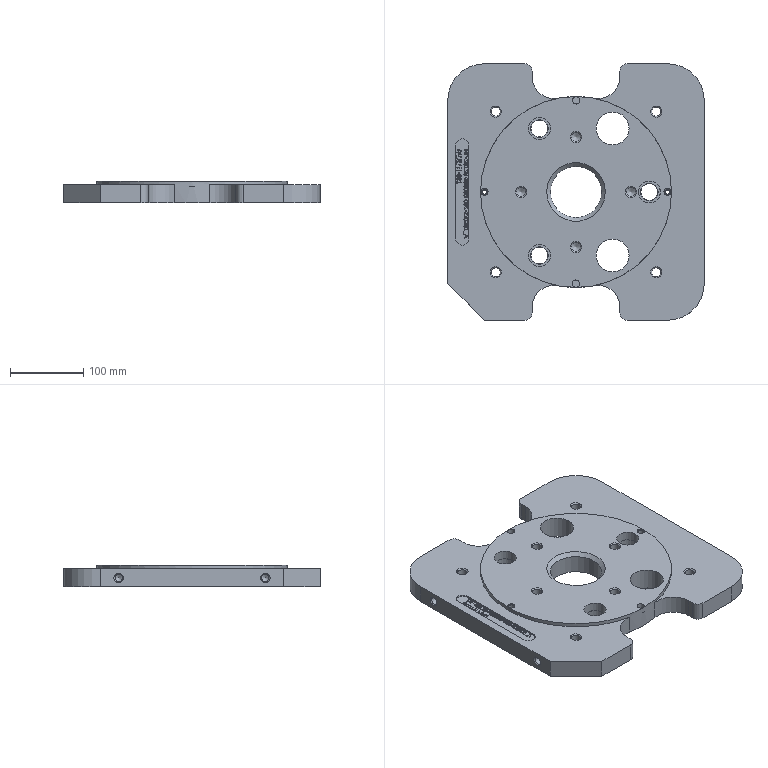CAM job | NX | mm | 3-axis | 4 set-ups | 62 operations | part box 350 x 350 x 30
set-up 1
1. Planar Milling | Mill Mill5 LX-D12 | PLANAR_MILLING_1 | path 52963.207 mm | 12.995 min
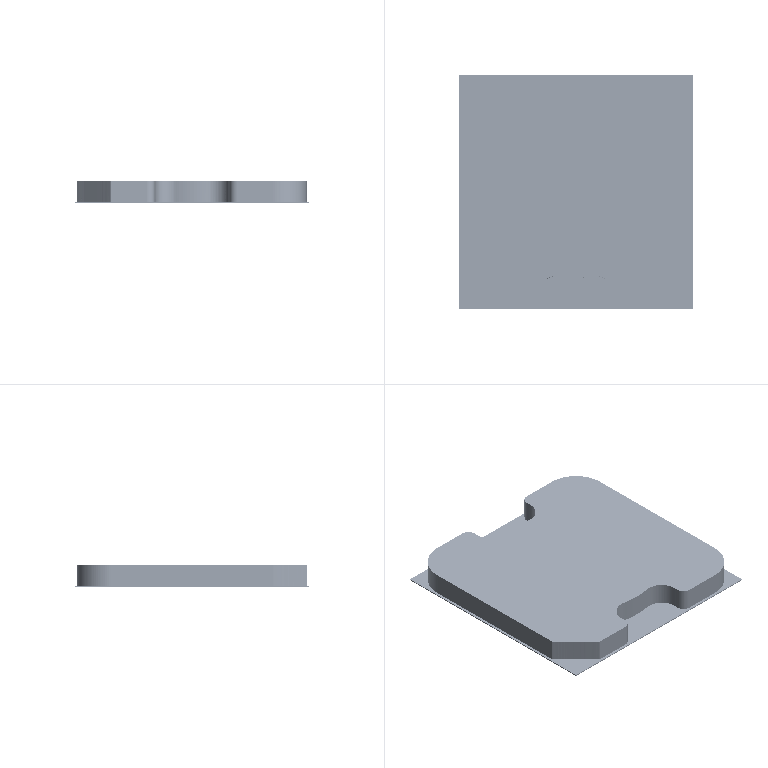2. Drilling | Mill MillChamfer DXZ-D6A90 | DRILLING_2 | path 472.41 mm | 0.166 min
3. Drilling | Drill DrillStandard ZT-D9.9 | DRILLING_3 | path 1885.71 mm | 2.188 min
4. Cavity Milling | Mill Mill5 LX-D12 | CAVITY_MILLING_4 | path 120910.672 mm | 30.327 min
5. Cavity Milling | Mill Mill5 LX-D12 | CAVITY_MILLING_5 | path 21409.338 mm | 17.162 min
set-up 2
6. Face Milling | Mill Mill5 E50R0.8 | FACE_MILLING_6 | path 20984.363 mm | 9.761 min
7. Planar Milling | Mill Mill5 LX-D12 | PLANAR_MILLING_7 | path 17688.841 mm | 4.155 min
8. Planar Milling | Mill Mill5 LX-D12 | PLANAR_MILLING_8 | path 2612.83 mm | 0.6251 min
9. Planar Milling | Mill Mill5 LX-D12 | PLANAR_MILLING_9 | path 3553.203 mm | 0.8071 min
10. Drilling | Mill MillChamfer DXZ-D6A90 | DRILLING_10 | path 344 mm | 0.1669 min
11. Drilling | Mill MillChamfer DXZ-D6A90 | DRILLING_11 | path 845.609 mm | 0.3496 min
12. Drilling | Drill DrillStandard ZT-D5.5 | DRILLING_12 | path 1324 mm | 1.534 min
13. Drilling | Drill DrillStandard ZT-D10.5 | DRILLING_13 | path 2815.498 mm | 3.098 min
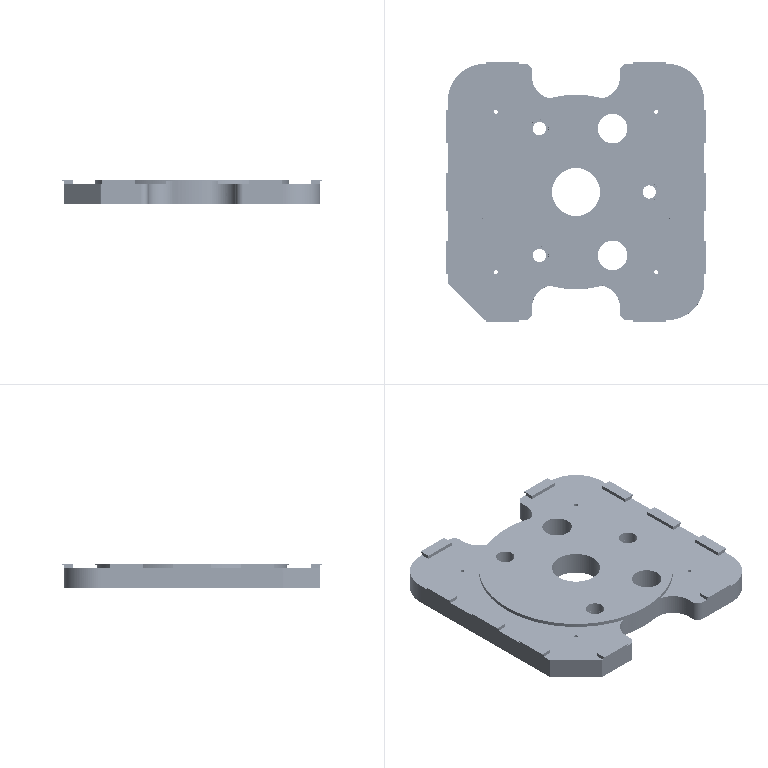14. Cylinder Milling | Mill Mill5 LX-D10 | CYLINDER_MILLING_14 | path 2394.779 mm | 1.918 min
15. Face Milling | Mill Mill5 E50R0.8 | FACE_MILLING_15 | path 6441 mm | 8.011 min
16. Cylinder Milling | Mill Mill5 LX-D10J | CYLINDER_MILLING_16 | path 1842.35 mm | 2.364 min
17. Planar Milling | Mill Mill5 LX-D12J | PLANAR_MILLING_17 | path 901.756 mm | 0.5999 min
18. Planar Milling | Mill Mill5 LX-D12J | PLANAR_MILLING_18 | path 3088.498 mm | 3.698 min
19. Thread Milling | Drill DrillThreadMill ST12X1.75-D10 | THREAD_MILLING_19 | path 4743.054 mm | 6.86 min
20. Thread Milling | Drill DrillThreadMill ST12X1.75-D10 | THREAD_MILLING_20 | path 1740.533 mm | 1.698 min
21. Volume Based 2.5D Milling | Mill MillChamfer DJ-D10A90 | VOLUME_BASED_2.5D_MILLING_21 | path 1306.051 mm | 0.5446 min
22. Fixed-axis Surface Contouring | Mill MillChamfer DJ-D10A90 | FIXED-AXIS_SURFACE_CONTOURING_22 | path 3704.367 mm | 2.34 min
23. Planar Milling | Mill Mill5 LX-D12J | PLANAR_MILLING_23 | path 13798.065 mm | 5.494 min
set-up 3
24. Face Milling | Mill Mill5 E50R0.8 | FACE_MILLING_24 | path 10729.483 mm | 5.016 min
25. Cavity Milling | Mill Mill5 LX-D12 | CAVITY_MILLING_25 | path 63705.335 mm | 15.092 min
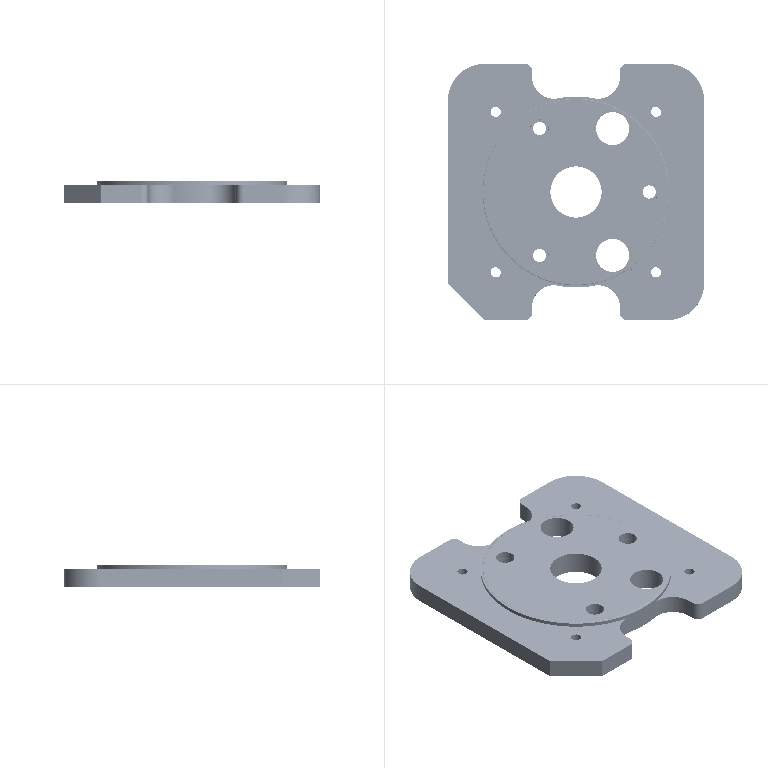26. Cylinder Milling | Mill Mill5 LX-D12 | CYLINDER_MILLING_26 | path 3593.116 mm | 3.95 min
27. Cylinder Milling | Mill Mill5 LX-D12 | CYLINDER_MILLING_27 | path 3455.636 mm | 3.694 min
28. Cylinder Milling | Mill Mill5 LX-D12 | CYLINDER_MILLING_28 | path 1601.601 mm | 1.295 min
29. Drilling | Mill MillChamfer DXZ-D6A90 | DRILLING_29 | path 739.906 mm | 0.3116 min
30. Drilling | Drill DrillStandard ZT-D11.5 | DRILLING_30 | path 1805.513 mm | 2.375 min
31. Drilling | Drill DrillStandard ZT-D7.5 | DRILLING_31 | path 598 mm | 0.7536 min
32. Cylinder Milling | Mill Mill5 LX-D8 | CYLINDER_MILLING_32 | path 2246.266 mm | 2.14 min
33. Volume Based 2.5D Milling | Mill Mill5 LX-D8 | VOLUME_BASED_2.5D_MILLING_33 | path 2636.289 mm | 0.7371 min
34. Cylinder Milling | Mill Mill5 LX-D6 | CYLINDER_MILLING_34 | path 689.766 mm | 0.4379 min
35. Cylinder Milling | Mill Mill5 LX-D6 | CYLINDER_MILLING_35 | path 721.625 mm | 0.5024 min
36. Face Milling | Mill Mill5 E50R0.8 | FACE_MILLING_36 | path 3024.894 mm | 3.736 min
37. Cylinder Milling | Mill Mill5 LX-D6J | CYLINDER_MILLING_37 | path 622.291 mm | 0.6705 min
38. Cylinder Milling | Mill Mill5 LX-D6J | CYLINDER_MILLING_38 | path 620.498 mm | 0.7172 min
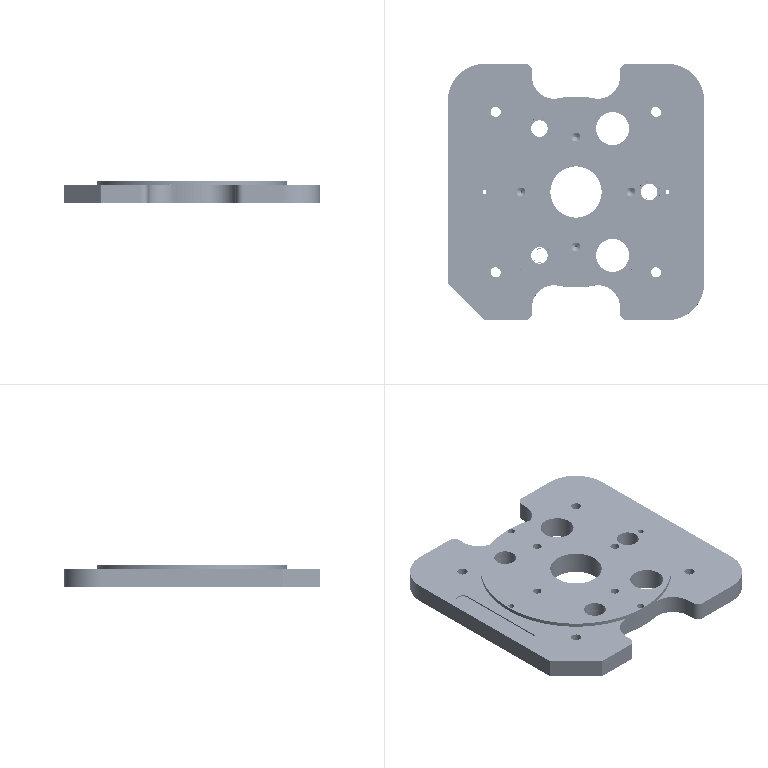39. Cylinder Milling | Mill Mill5 LX-D8J | CYLINDER_MILLING_39 | path 2076.707 mm | 3.799 min
40. Volume Based 2.5D Milling | Mill Mill5 LX-D8J | VOLUME_BASED_2.5D_MILLING_40 | path 817.628 mm | 1.033 min
41. Volume Based 2.5D Milling | Mill Mill5 LX-D8J | VOLUME_BASED_2.5D_MILLING_41 | path 348.948 mm | 0.3741 min
42. Volume Based 2.5D Milling | Mill Mill5 LX-D12J | VOLUME_BASED_2.5D_MILLING_42 | path 11476.04 mm | 12.766 min
43. Volume Based 2.5D Milling | Mill Mill5 LX-D12J | VOLUME_BASED_2.5D_MILLING_43 | path 918.725 mm | 0.9751 min
44. Cylinder Milling | Mill Mill5 LX-D12J | CYLINDER_MILLING_44 | path 1948.545 mm | 3.739 min
45. Cylinder Milling | Mill Mill5 LX-D12J | CYLINDER_MILLING_45 | path 1934.602 mm | 3.527 min
46. Cylinder Milling | Mill Mill5 LX-D12J | CYLINDER_MILLING_46 | path 1094.948 mm | 1.218 min
47. Planar Milling | Mill Mill5 LX-D12J | PLANAR_MILLING_47 | path 515.038 mm | 0.487 min
48. Volume Based 2.5D Milling | Mill MillChamfer DJ-D12A90 | VOLUME_BASED_2.5D_MILLING_48 | path 961.193 mm | 0.9166 min
49. Volume Based 2.5D Milling | Mill MillChamfer DJ-D12A90 | VOLUME_BASED_2.5D_MILLING_49 | path 1365.965 mm | 0.9176 min
50. Volume Based 2.5D Milling | Mill MillChamfer DJ-D12A90 | VOLUME_BASED_2.5D_MILLING_50 | path 737.716 mm | 0.4306 min
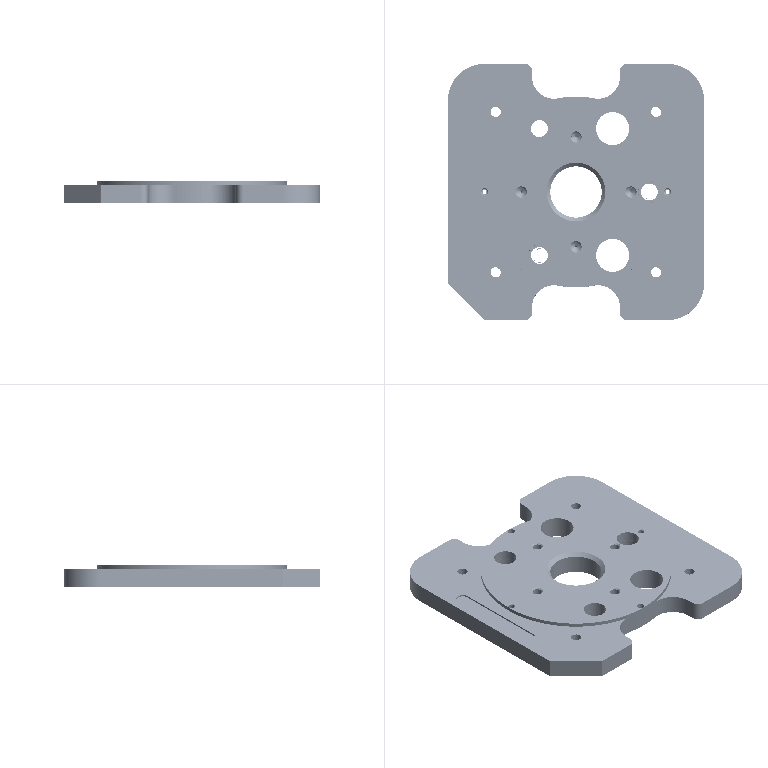51. Volume Based 2.5D Milling | Mill MillChamfer DJ-D12A90 | VOLUME_BASED_2.5D_MILLING_51 | path 1734.442 mm | 0.9544 min
52. Volume Based 2.5D Milling | Mill MillChamfer DJ-D12A90 | VOLUME_BASED_2.5D_MILLING_52 | path 857.35 mm | 0.2619 min
53. Thread Milling | Drill DrillThreadMill ST12X1.75-D10 | THREAD_MILLING_53 | path 3047.876 mm | 4.493 min
54. Thread Milling | Drill DrillThreadMill ST12X1.75-D10 | THREAD_MILLING_54 | path 1221.368 mm | 1.346 min
55. Planar Text | Mill Mill5 KZ-D0.5R0.25 | PLANAR_TEXT_55 | path 3465.088 mm | 1.493 min
56. Planar Text | Mill Mill5 KZ-D0.5R0.25 | PLANAR_TEXT_56 | path 285.843 mm | 0.1204 min
57. Planar Milling | Mill Mill5 LX-D12J | PLANAR_MILLING_57 | path 3124.934 mm | 1.531 min
set-up 4
58. Drilling | Mill MillChamfer DXZ-D6A90 | DRILLING_58 | path 284 mm | 0.1076 min
59. Drilling | Drill DrillStandard ZT-D10.3 | DRILLING_59 | path 1029.012 mm | 1.069 min
60. Volume Based 2.5D Milling | Mill MillChamfer DJ-D6A90 | VOLUME_BASED_2.5D_MILLING_60 | path 485.736 mm | 0.2353 min
61. Thread Milling | Drill DrillThreadMill M12X1.75-D10_ | THREAD_MILLING_61 | path 1031.904 mm | 1.147 min
62. Thread Milling | Drill DrillThreadMill M12X1.75-D10_ | THREAD_MILLING_62 | path 474.213 mm | 0.3475 min